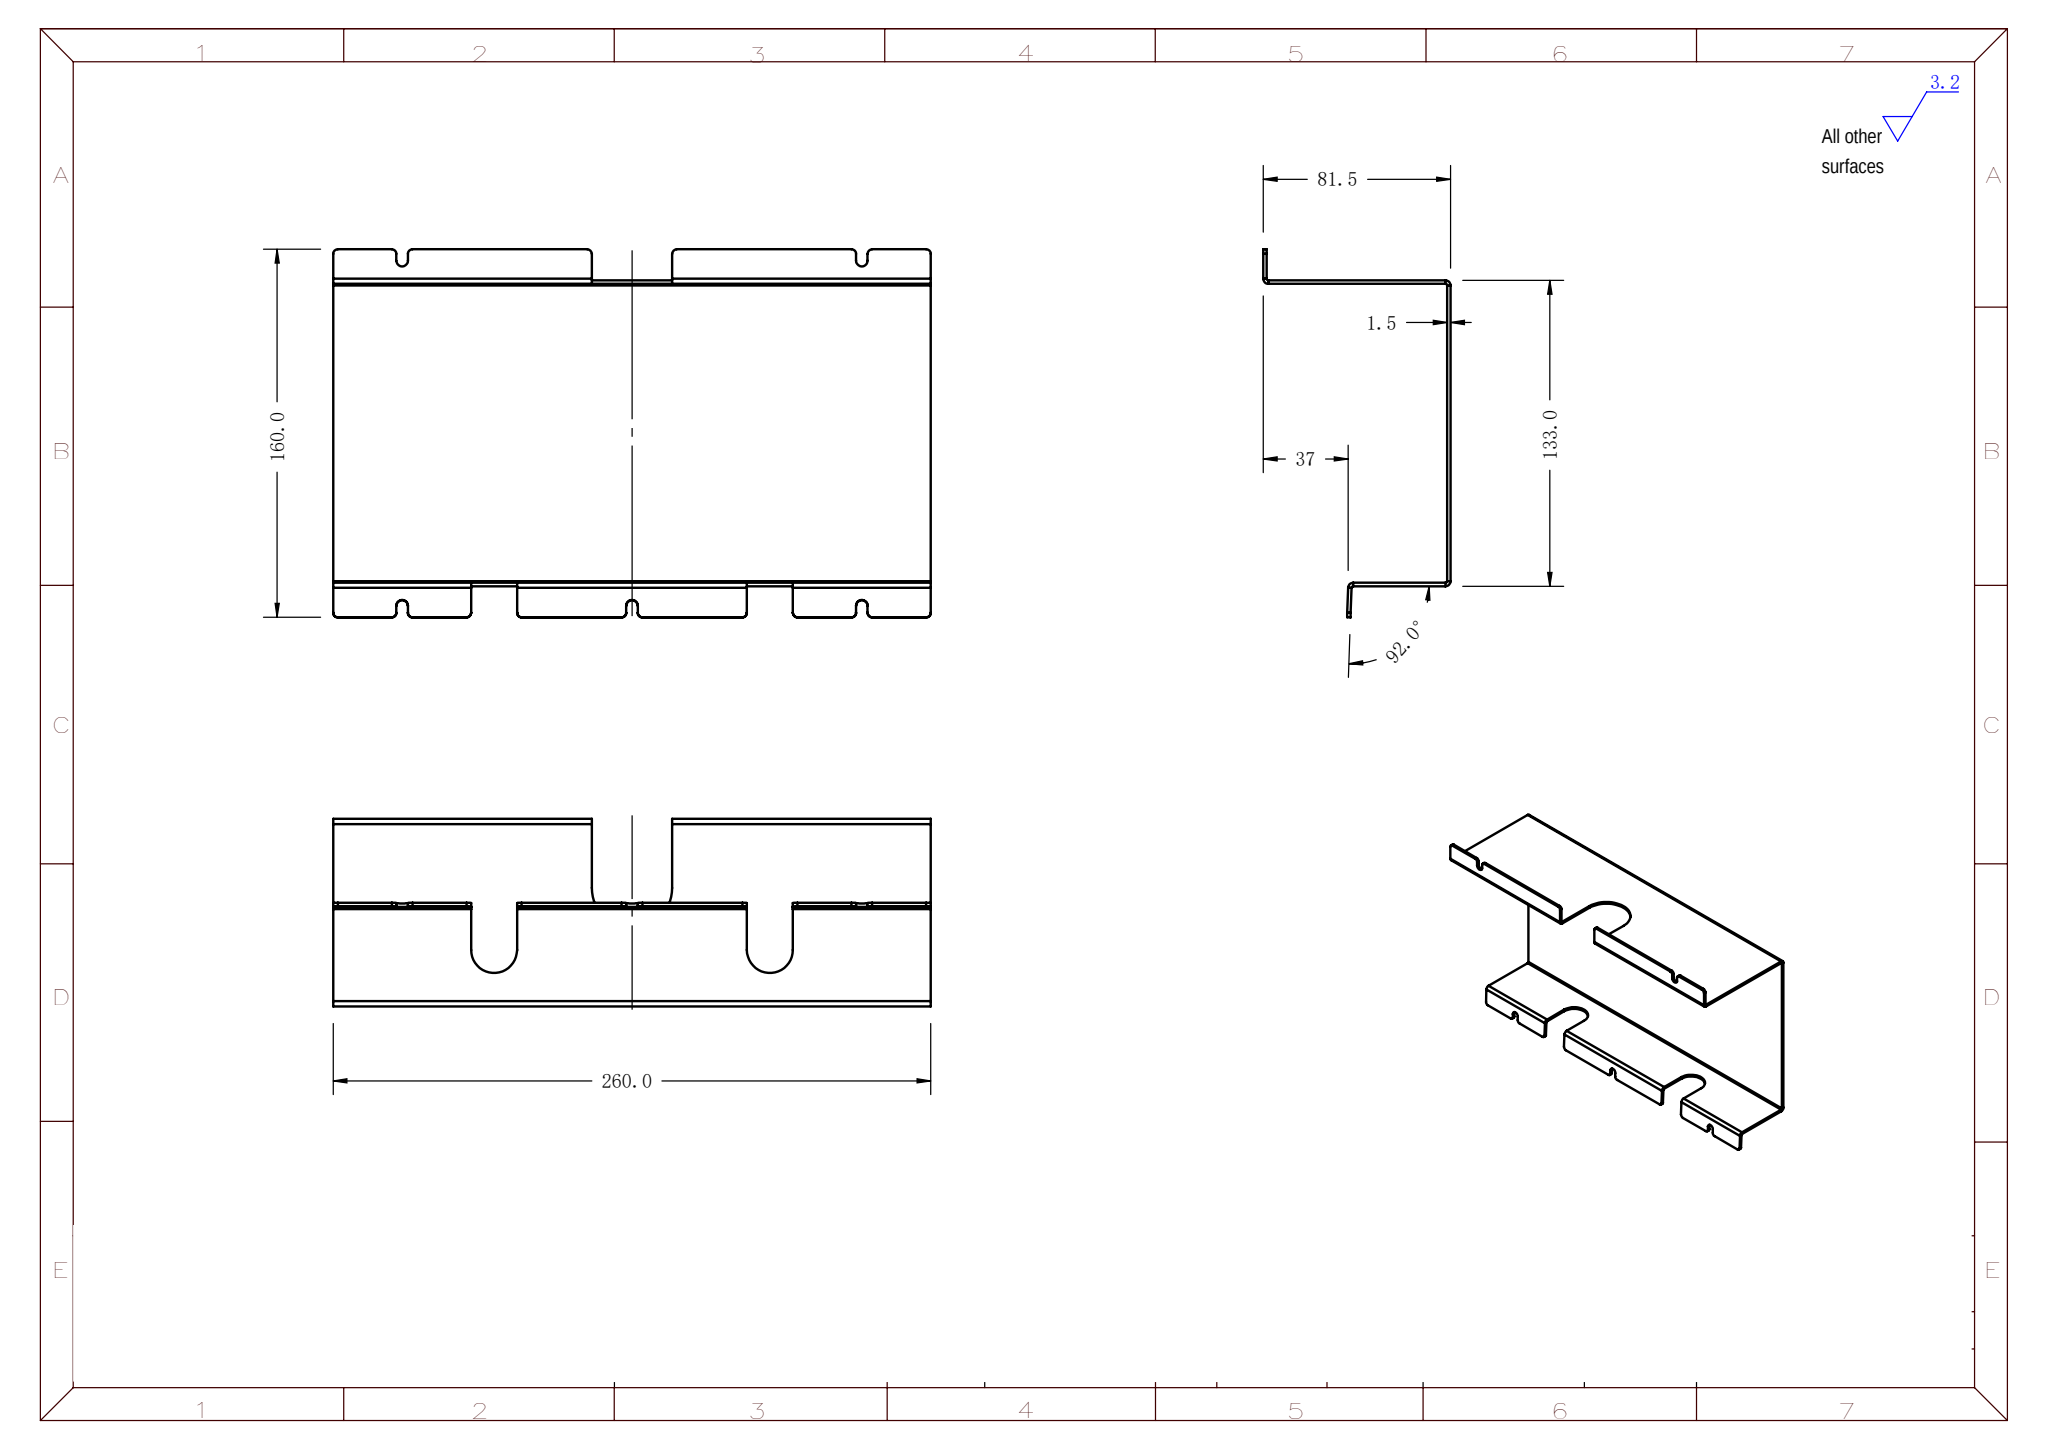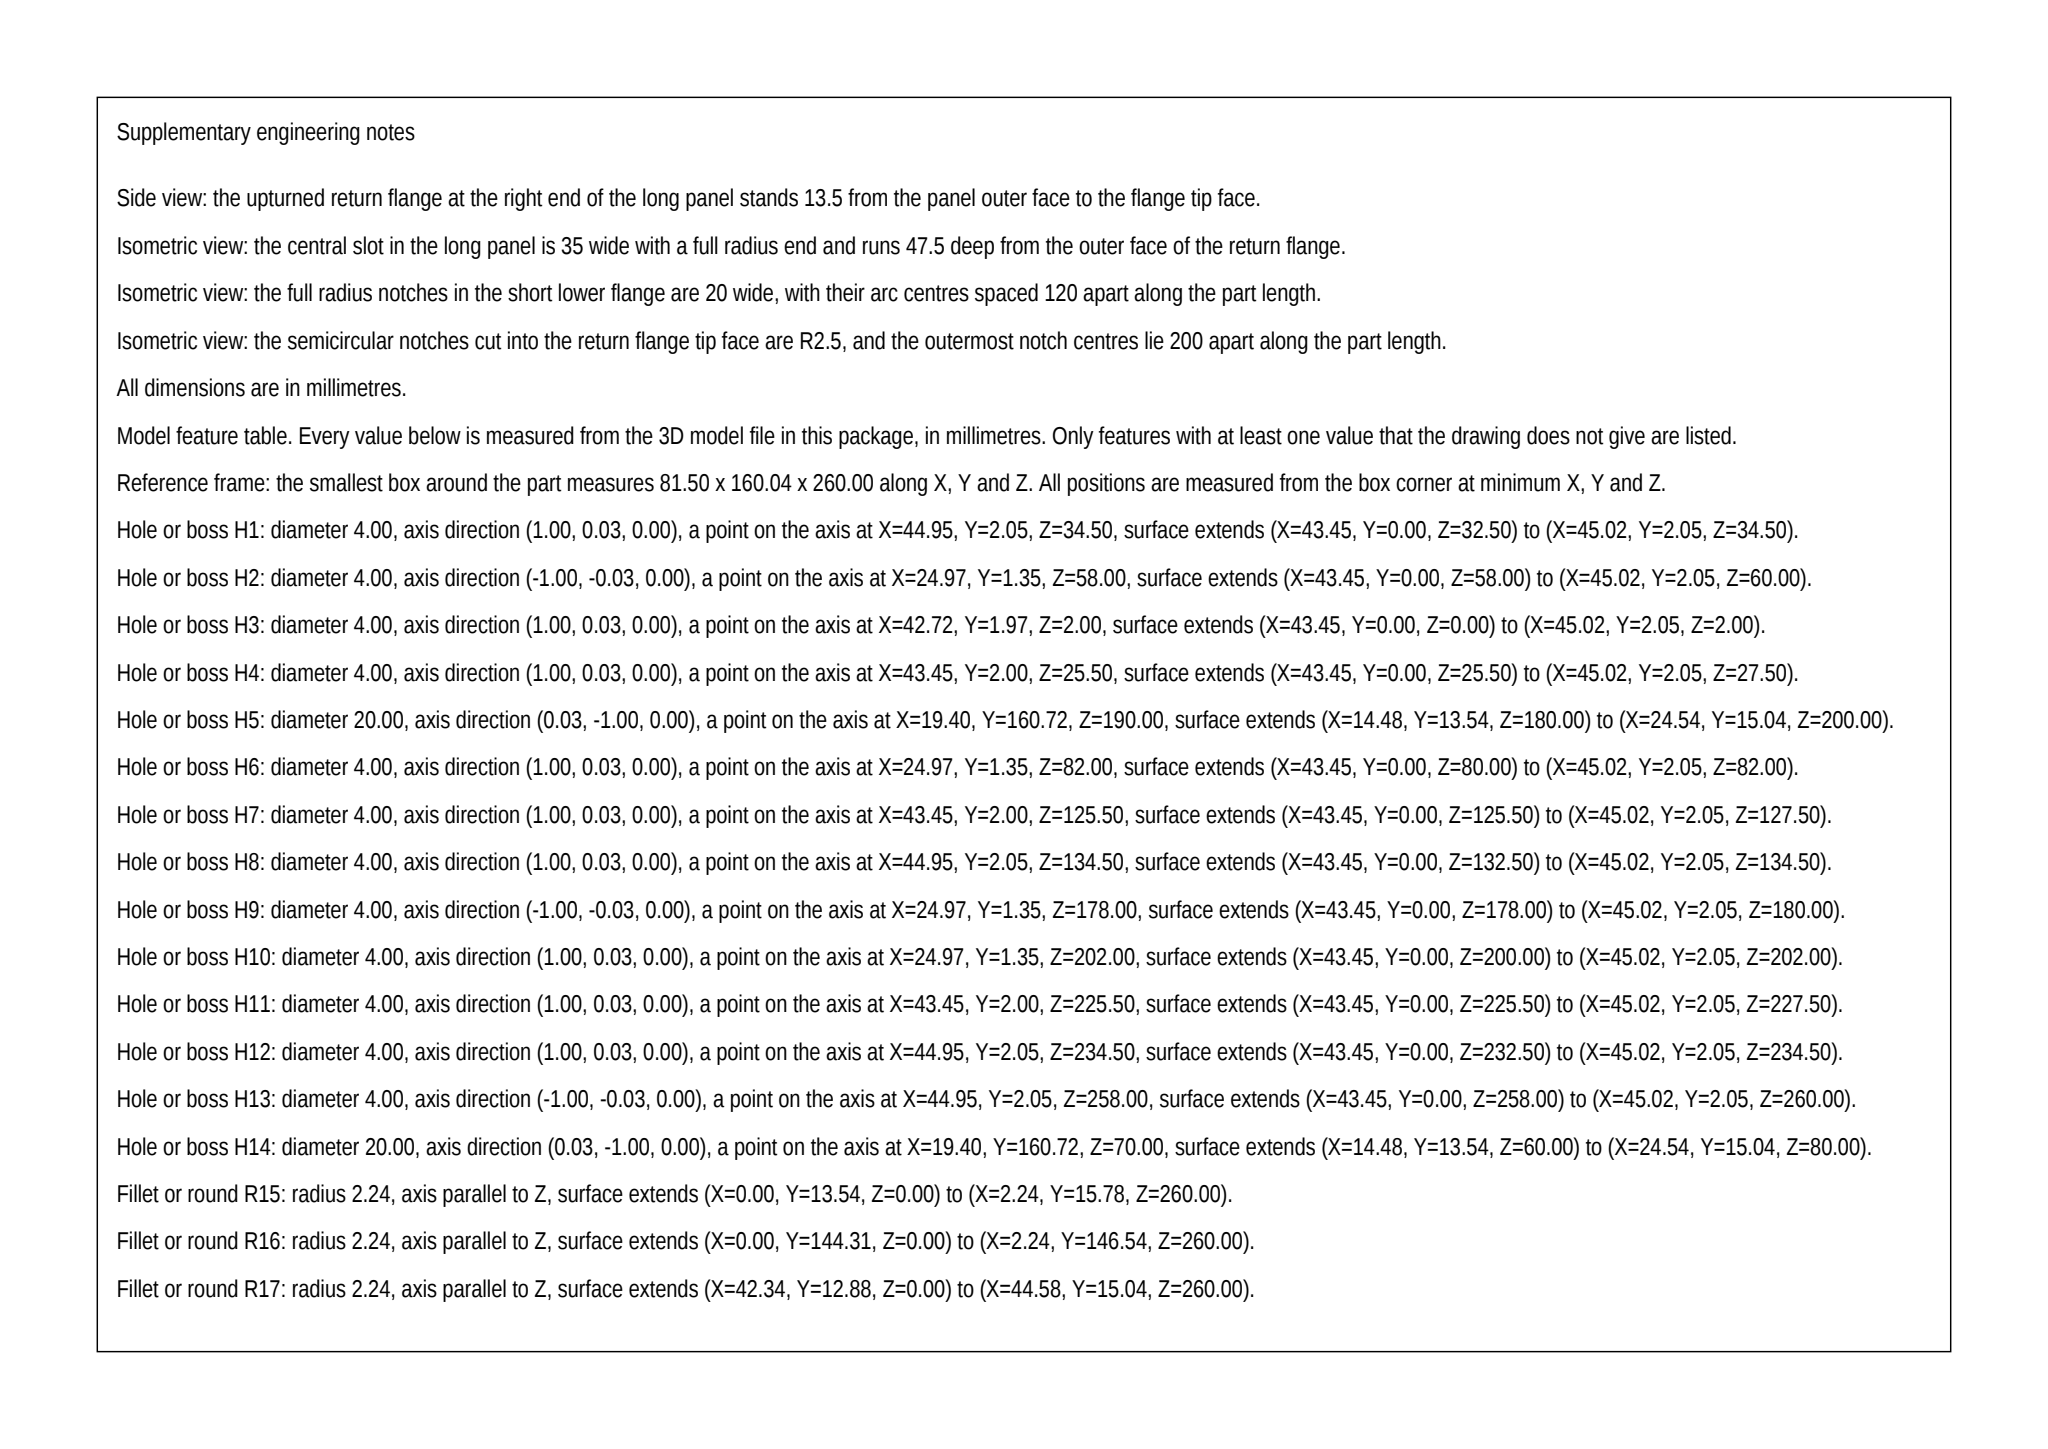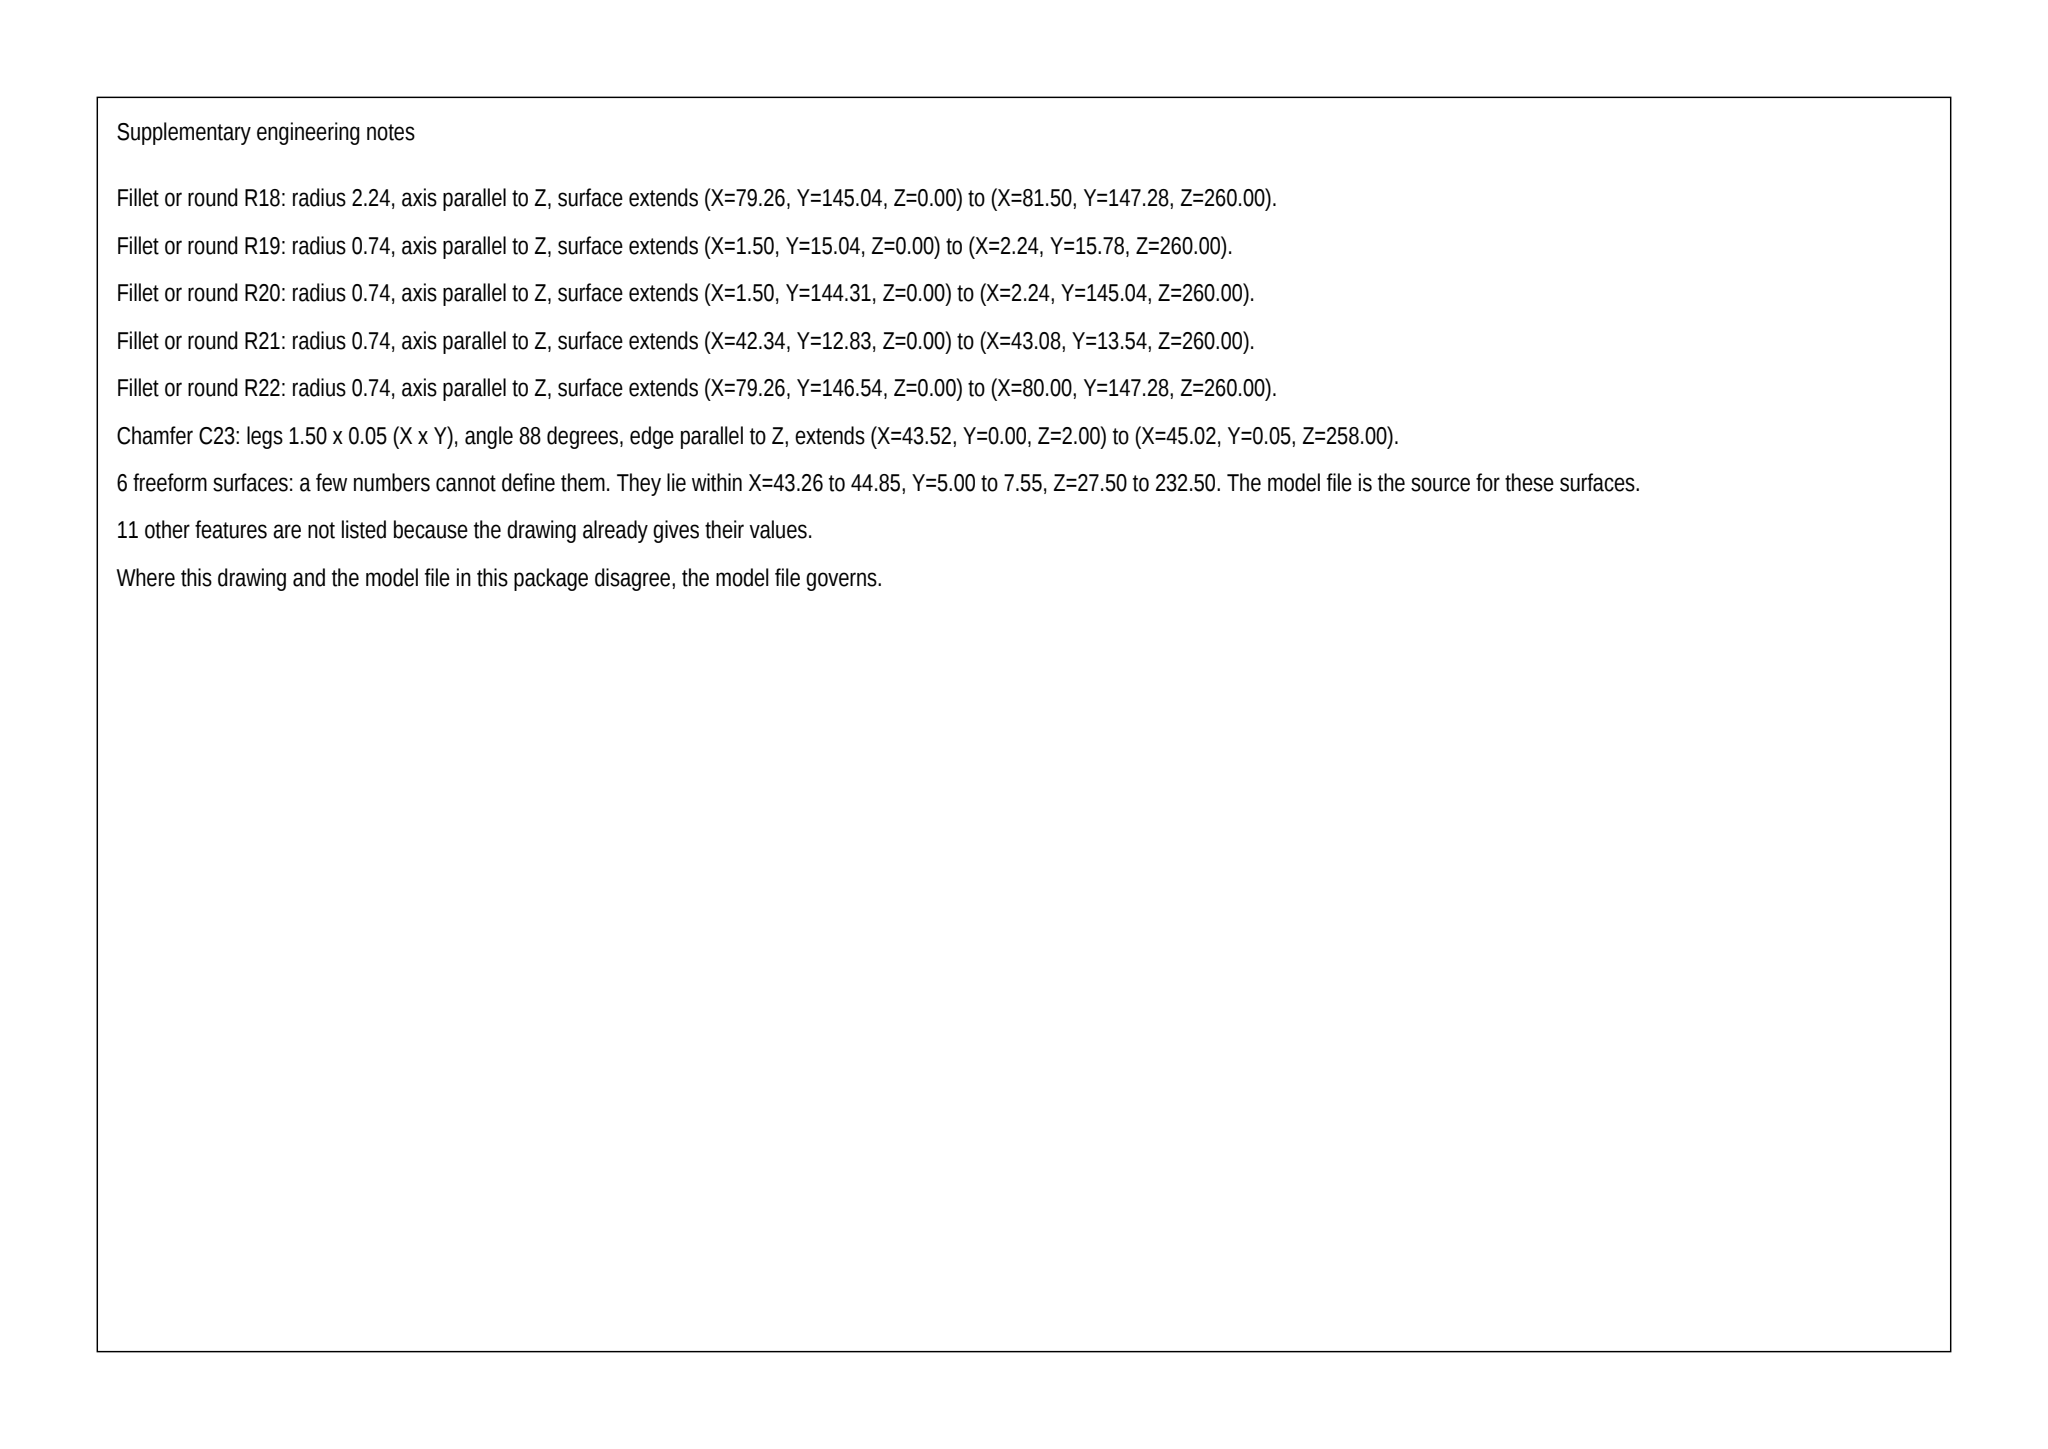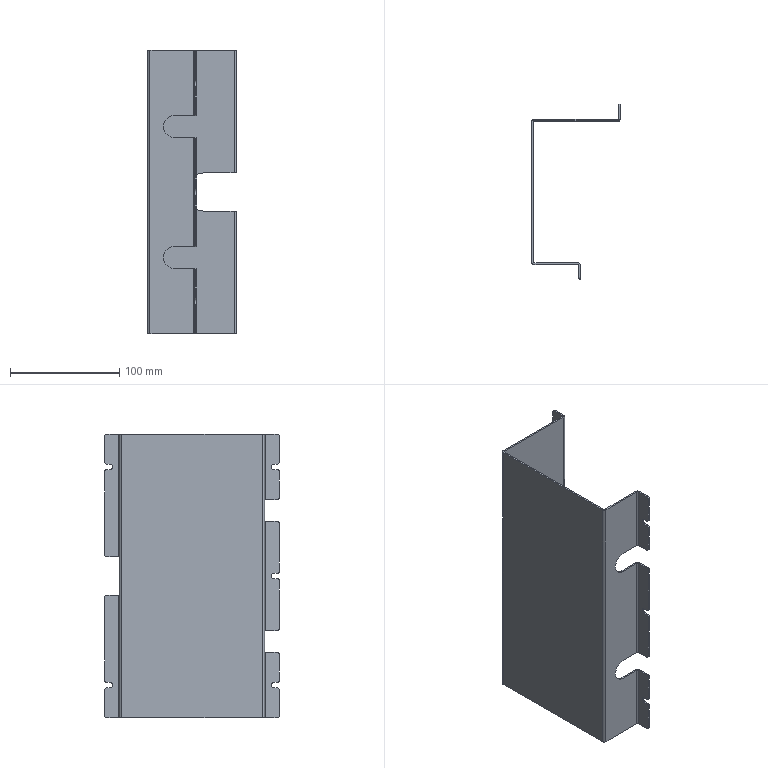Part | SolidWorks | mm | 1 solid | 109 faces | box 81.5 x 160.04 x 260 mm | volume 103708 mm3 | plane 64 | cylinder 39 | spline 6 | commonest cylinder face diameters 4 x20 1.473 x7 4.473 x7 5 x2 20 x2 35 x1